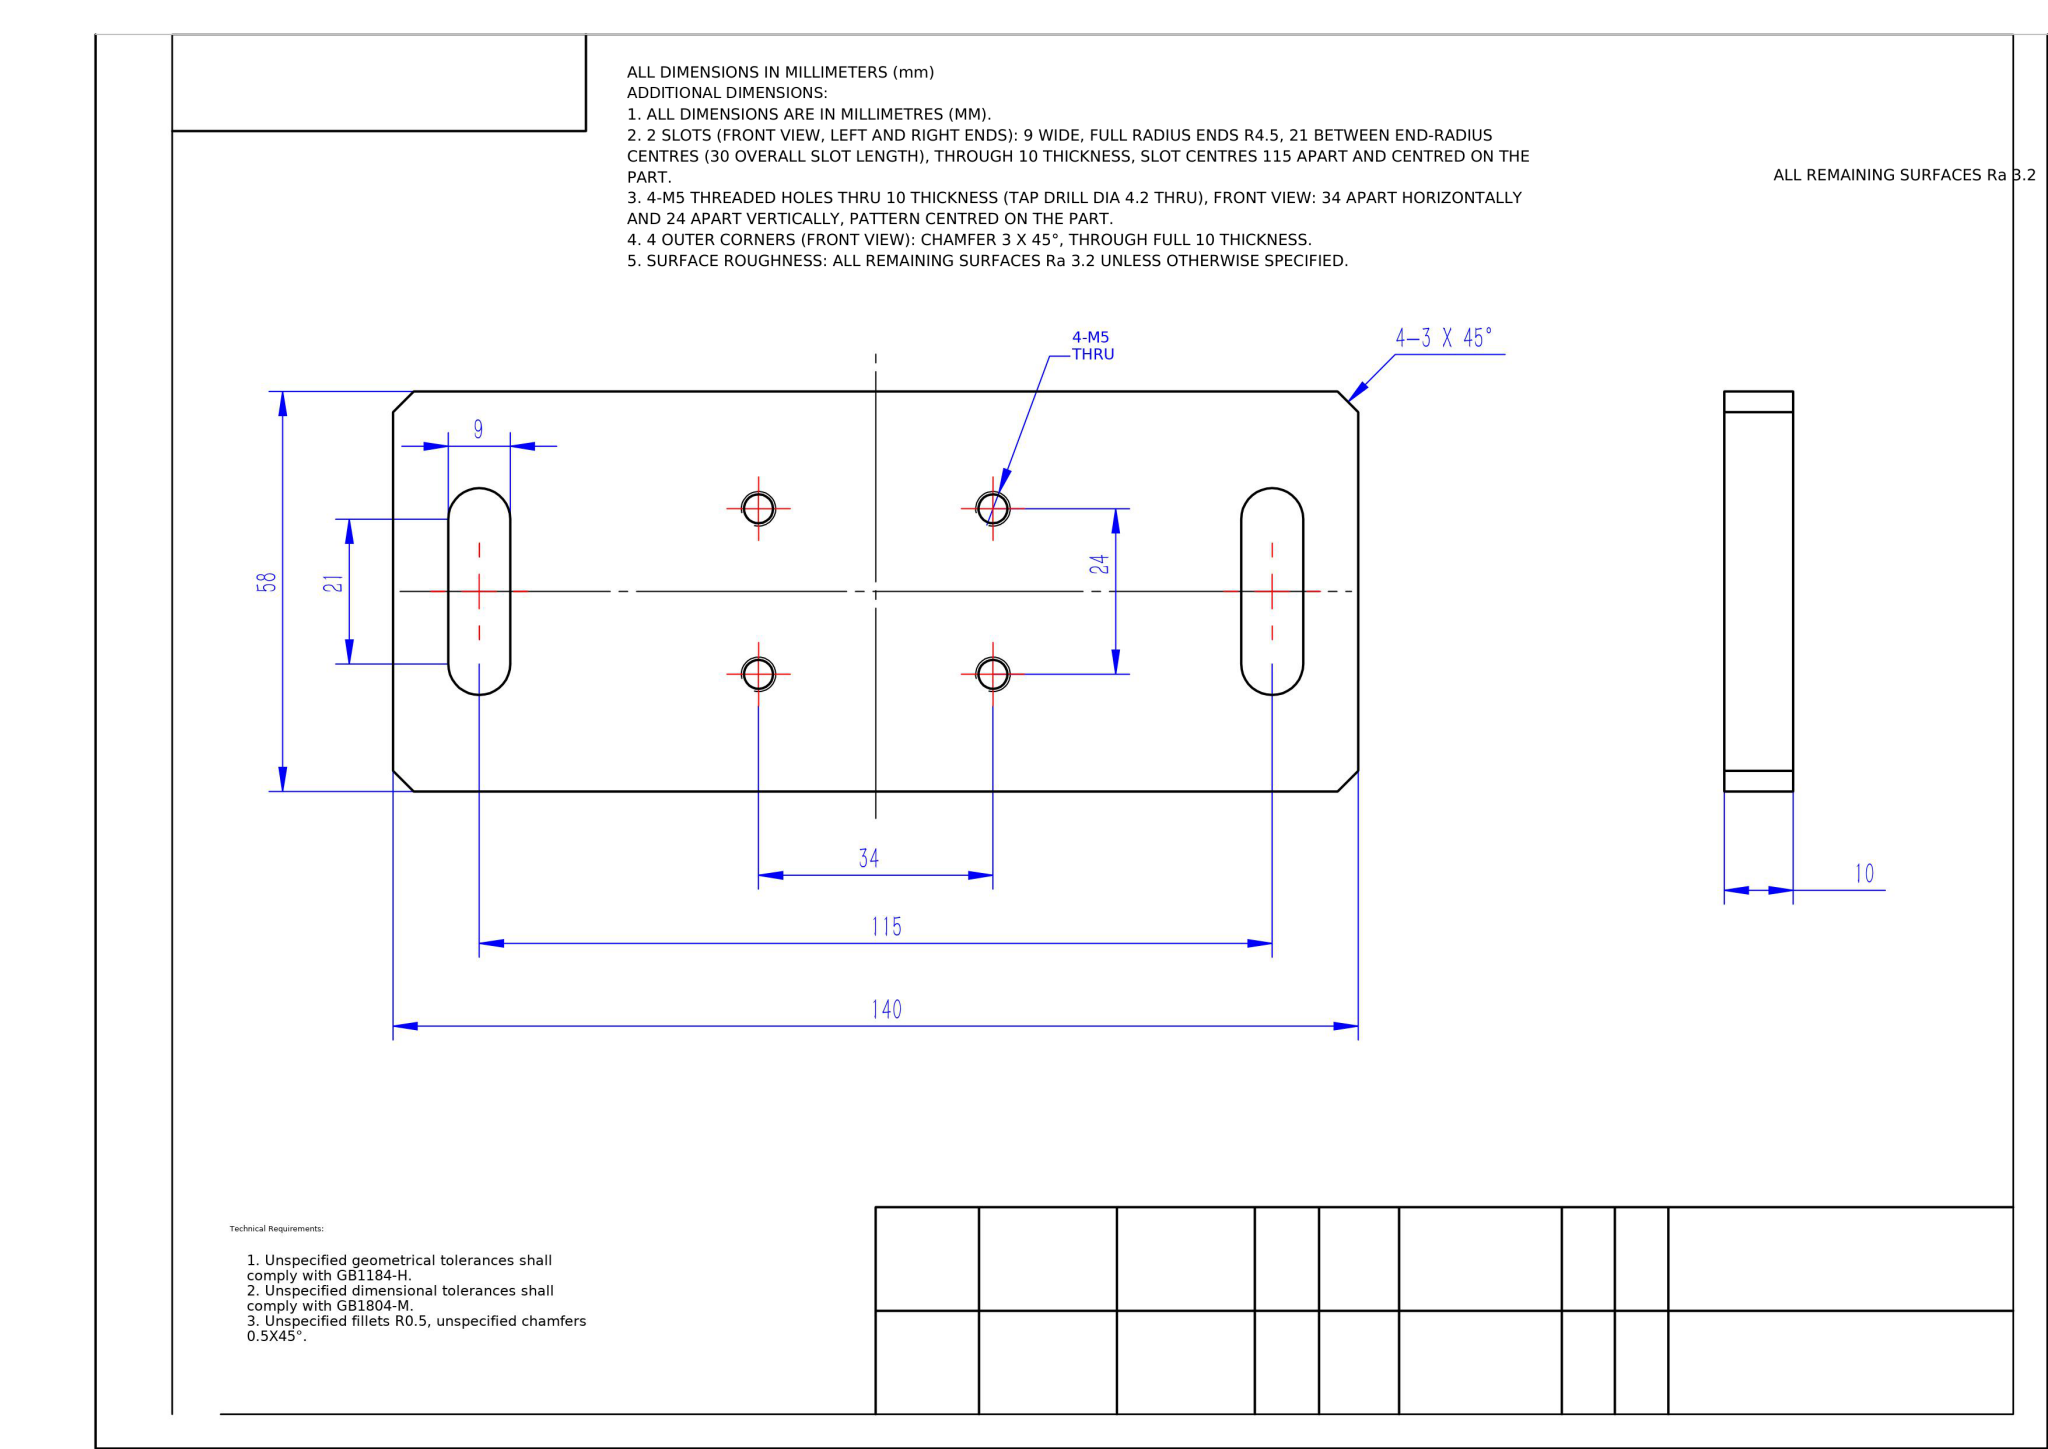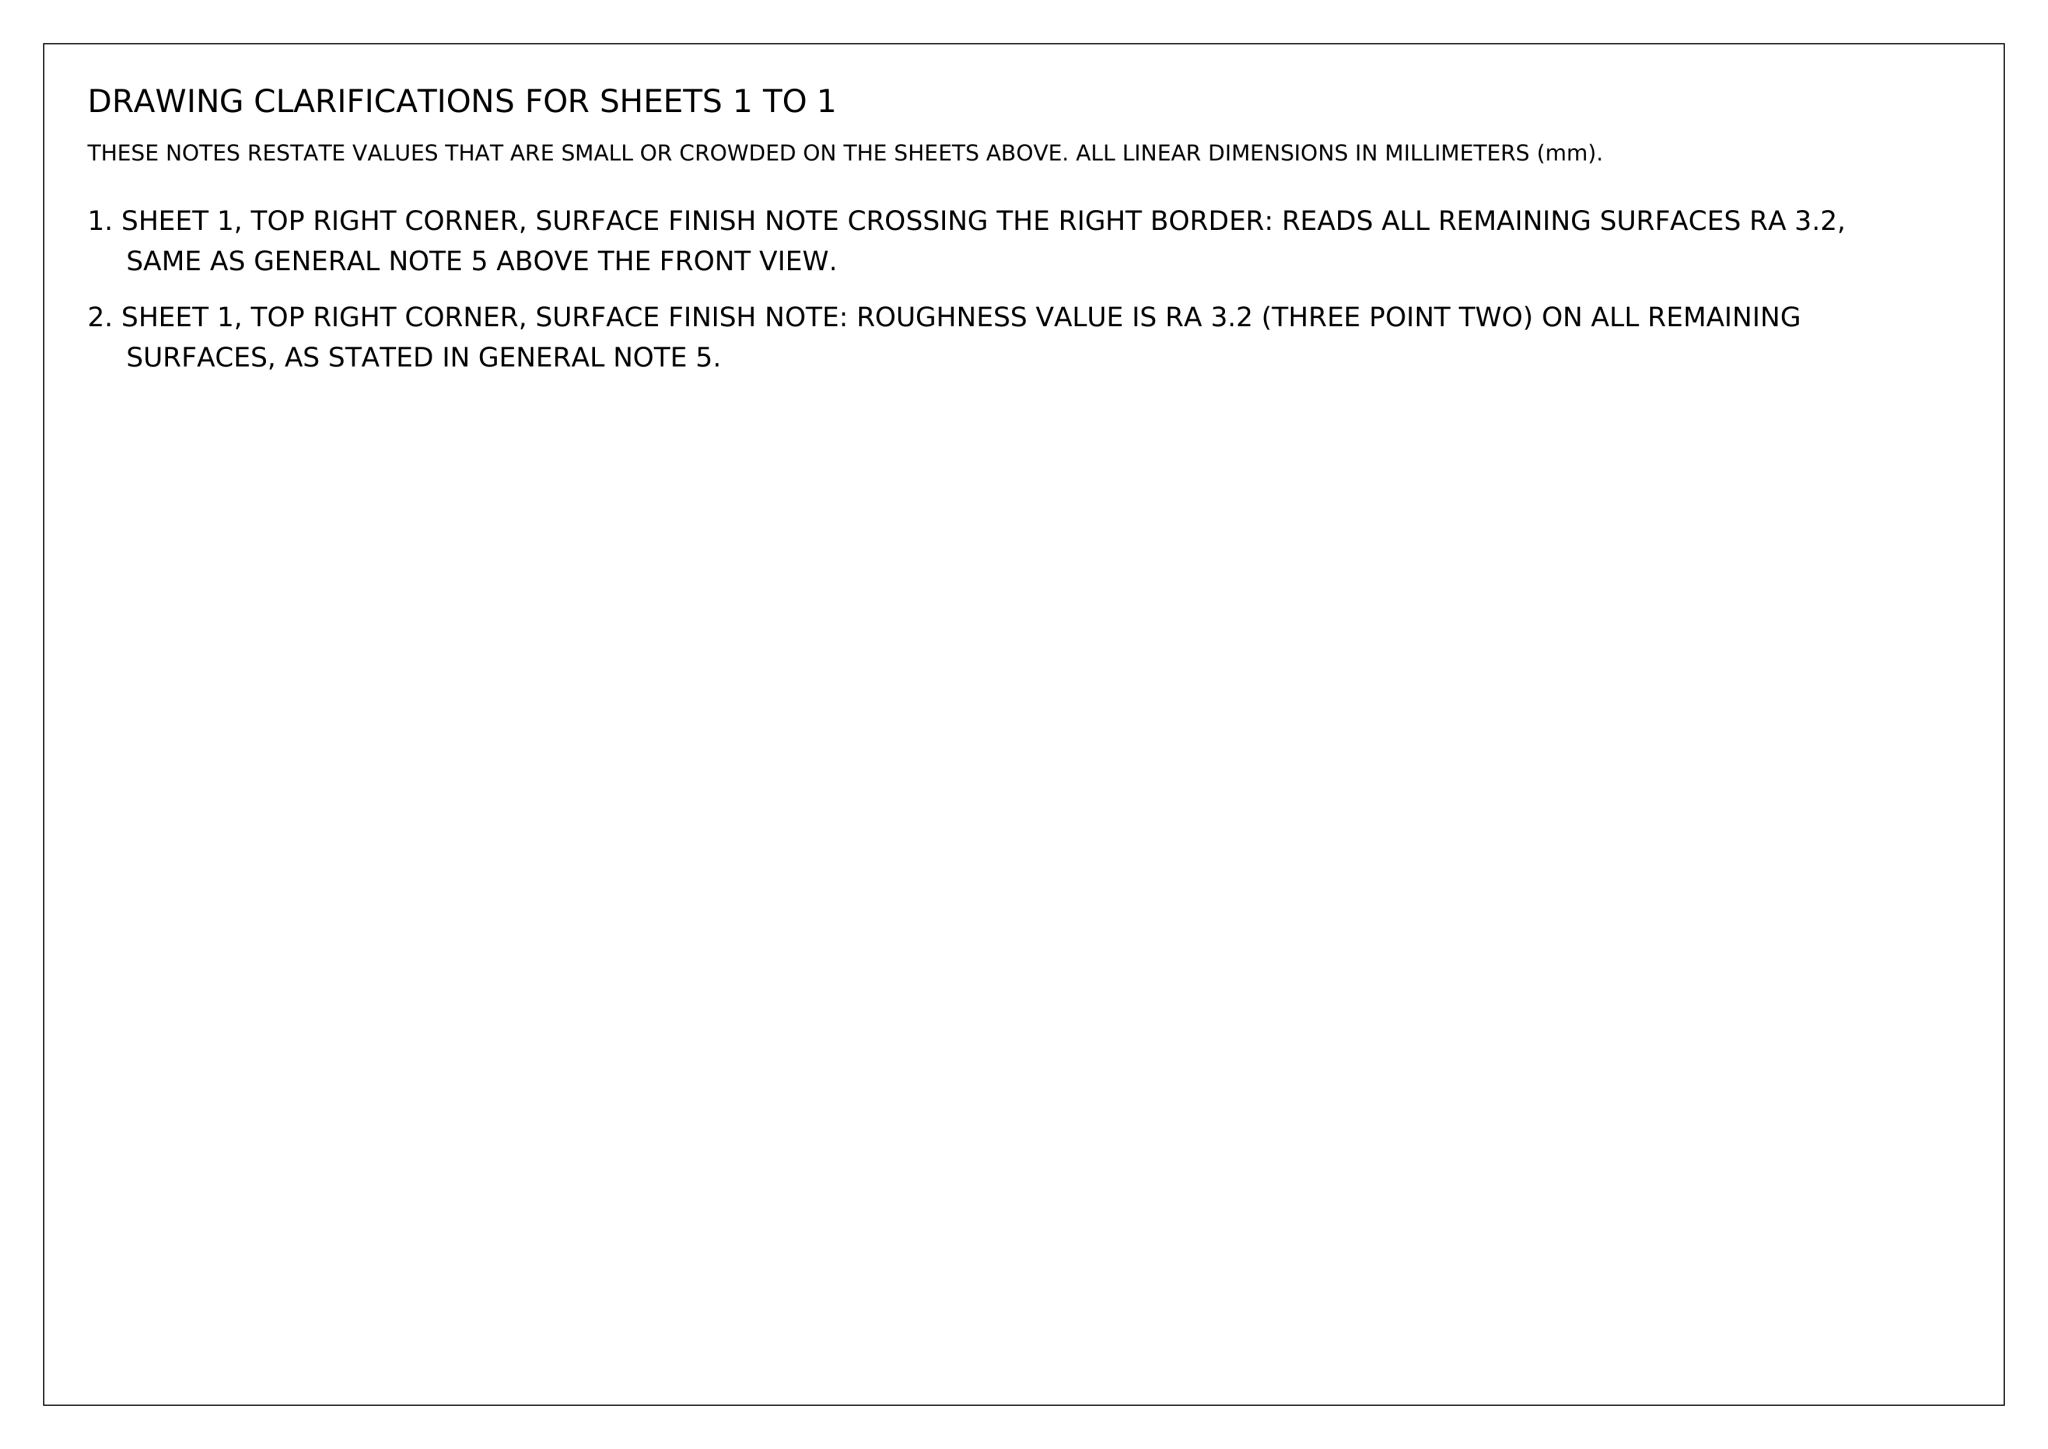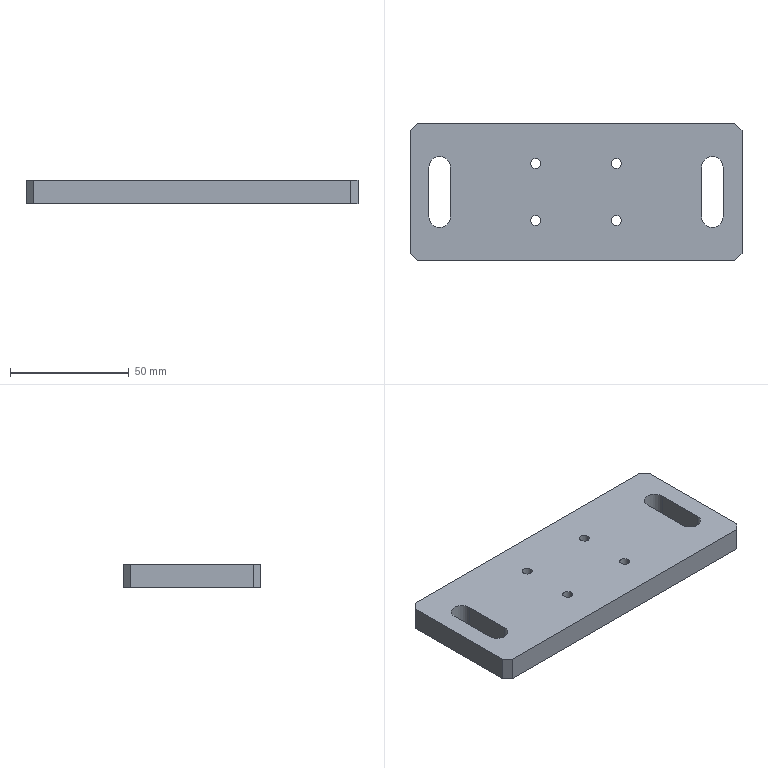Part | NX | mm | 1 solid | 26 faces | box 140 x 58 x 10 mm | volume 75413 mm3 | plane 14 | cylinder 12 | commonest cylinder face diameters 4.2 x8 9 x4